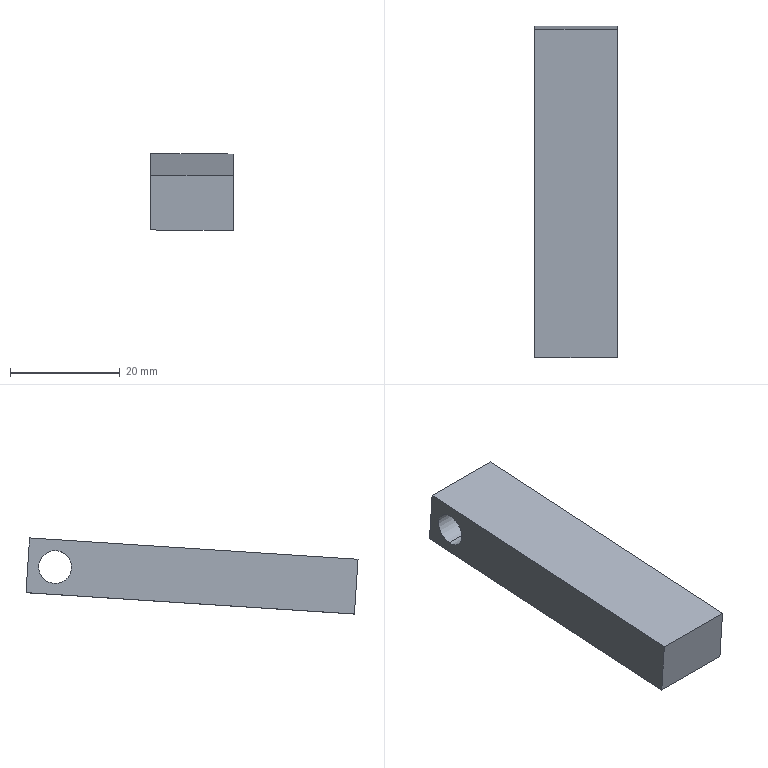Component | SolidWorks | ClampingPlate-1 | 1 solid | 8 faces | box 15.01 x 60.52 x 13.88 mm | volume 8576 mm3 | plane 6 | cylinder 2 | commonest cylinder face diameters 6 x2
build123d program:
from build123d import *

# Parameters (mm, degrees)
SKETCH1_W           = 60
SKETCH1_H           = 10
BOSS_EXTRUDE1_DEPTH = 15
SKETCH2_R           = 3
CUT_EXTRUDE1_DEPTH  = 20


with BuildPart() as part:
    # Sketch1 → Boss-Extrude1 (new body)
    with BuildSketch(Plane(origin=(0, 0, 0), x_dir=(1, 0, 0), z_dir=(0, 1, 0))):
        Rectangle(SKETCH1_W, SKETCH1_H)
    extrude(amount=BOSS_EXTRUDE1_DEPTH)

    # Sketch2 → Cut-Extrude1 (cut)
    with BuildSketch(Plane(origin=(0, 15, 0), x_dir=(1, 0, 0), z_dir=(0, 1, 0))):
        with Locations(Location((25, 0, 0), (0, 0, 270))):
            Circle(SKETCH2_R)
    extrude(amount=-CUT_EXTRUDE1_DEPTH, mode=Mode.SUBTRACT)


solid = part.part

# Placed as in the assembly
solid = solid.moved(Location((-132.643, 740.362, 1090.615), (3.717, 0.06177, 89.996)))
STEP:
#1=CARTESIAN_POINT('',(-5.222,30.123,43.119));
#2=VERTEX_POINT('',#1);
#3=CARTESIAN_POINT('',(-5.222,30.138,42.884));
#4=VERTEX_POINT('',#3);
#5=CARTESIAN_POINT('',(-5.222,30.13,43.001));
#6=DIRECTION('',(1.,0.,-0.00108));
#7=DIRECTION('',(-0.001078,0.06482,-0.9979));
#8=AXIS2_PLACEMENT_3D('',#5,#6,#7);
#9=CIRCLE('',#8,0.1181);
#10=EDGE_CURVE('',#2,#4,#9,.T.);
#11=ORIENTED_EDGE('',*,*,#10,.T.);
#12=CARTESIAN_POINT('',(-5.813,30.138,42.884));
#13=VERTEX_POINT('',#12);
#14=CARTESIAN_POINT('',(-5.025,30.138,42.883));
#15=DIRECTION('',(-1.,-0.,0.00108));
#16=VECTOR('',#15,39.37);
#17=LINE('',#14,#16);
#18=EDGE_CURVE('',#4,#13,#17,.T.);
#19=ORIENTED_EDGE('',*,*,#18,.T.);
#20=CARTESIAN_POINT('',(-5.813,30.123,43.12));
#21=VERTEX_POINT('',#20);
#22=CARTESIAN_POINT('',(-5.813,30.13,43.002));
#23=DIRECTION('',(-1.,-0.,0.00108));
#24=DIRECTION('',(0.001078,-0.06482,0.9979));
#25=AXIS2_PLACEMENT_3D('',#22,#23,#24);
#26=CIRCLE('',#25,0.1181);
#27=EDGE_CURVE('',#13,#21,#26,.T.);
#28=ORIENTED_EDGE('',*,*,#27,.T.);
#29=CARTESIAN_POINT('',(-5.025,30.123,43.119));
#30=DIRECTION('',(-1.,-0.,0.00108));
#31=VECTOR('',#30,39.37);
#32=LINE('',#29,#31);
#33=EDGE_CURVE('',#2,#21,#32,.T.);
#34=ORIENTED_EDGE('',*,*,#33,.F.);
#35=EDGE_LOOP('',(#11,#19,#28,#34));
#36=FACE_OUTER_BOUND('',#35,.T.);
#37=CARTESIAN_POINT('',(-5.025,30.13,43.001));
#38=DIRECTION('',(-1.,-0.,0.00108));
#39=DIRECTION('',(0.001078,-0.06482,0.9979));
#40=AXIS2_PLACEMENT_3D('',#37,#38,#39);
#41=CYLINDRICAL_SURFACE('',#40,0.1181);
#42=ADVANCED_FACE('',(#36),#41,.F.);
#43=CARTESIAN_POINT('',(-5.222,30.314,43.211));
#44=VERTEX_POINT('',#43);
#45=CARTESIAN_POINT('',(-5.222,30.339,42.818));
#46=VERTEX_POINT('',#45);
#47=CARTESIAN_POINT('',(-5.222,30.314,43.211));
#48=DIRECTION('',(-0.001078,0.06482,-0.9979));
#49=VECTOR('',#48,39.37);
#50=LINE('',#47,#49);
#51=EDGE_CURVE('',#44,#46,#50,.T.);
#52=ORIENTED_EDGE('',*,*,#51,.T.);
#53=CARTESIAN_POINT('',(-5.813,30.339,42.818));
#54=VERTEX_POINT('',#53);
#55=CARTESIAN_POINT('',(-5.813,30.339,42.818));
#56=DIRECTION('',(1.,0.,-0.00108));
#57=VECTOR('',#56,39.37);
#58=LINE('',#55,#57);
#59=EDGE_CURVE('',#54,#46,#58,.T.);
#60=ORIENTED_EDGE('',*,*,#59,.F.);
#61=CARTESIAN_POINT('',(-5.812,30.314,43.211));
#62=VERTEX_POINT('',#61);
#63=CARTESIAN_POINT('',(-5.812,30.314,43.211));
#64=DIRECTION('',(-0.001078,0.06482,-0.9979));
#65=VECTOR('',#64,39.37);
#66=LINE('',#63,#65);
#67=EDGE_CURVE('',#62,#54,#66,.T.);
#68=ORIENTED_EDGE('',*,*,#67,.F.);
#69=CARTESIAN_POINT('',(-5.812,30.314,43.211));
#70=DIRECTION('',(1.,0.,-0.00108));
#71=VECTOR('',#70,39.37);
#72=LINE('',#69,#71);
#73=EDGE_CURVE('',#62,#44,#72,.T.);
#74=ORIENTED_EDGE('',*,*,#73,.T.);
#75=EDGE_LOOP('',(#52,#60,#68,#74));
#76=FACE_OUTER_BOUND('',#75,.T.);
#77=CARTESIAN_POINT('',(-5.812,30.314,43.211));
#78=DIRECTION('',(-0.00007004,-0.9979,-0.06482));
#79=DIRECTION('',(0.001078,-0.06482,0.9979));
#80=AXIS2_PLACEMENT_3D('',#77,#78,#79);
#81=PLANE('',#80);
#82=ADVANCED_FACE('',(#76),#81,.F.);
#83=CARTESIAN_POINT('',(-5.222,27.982,42.665));
#84=VERTEX_POINT('',#83);
#85=CARTESIAN_POINT('',(-5.222,27.982,42.665));
#86=DIRECTION('',(-0.00007004,-0.9979,-0.06482));
#87=VECTOR('',#86,39.37);
#88=LINE('',#85,#87);
#89=EDGE_CURVE('',#46,#84,#88,.T.);
#90=ORIENTED_EDGE('',*,*,#89,.T.);
#91=CARTESIAN_POINT('',(-5.813,27.982,42.665));
#92=VERTEX_POINT('',#91);
#93=CARTESIAN_POINT('',(-5.813,27.982,42.665));
#94=DIRECTION('',(1.,0.,-0.00108));
#95=VECTOR('',#94,39.37);
#96=LINE('',#93,#95);
#97=EDGE_CURVE('',#92,#84,#96,.T.);
#98=ORIENTED_EDGE('',*,*,#97,.F.);
#99=CARTESIAN_POINT('',(-5.813,27.982,42.665));
#100=DIRECTION('',(-0.00007004,-0.9979,-0.06482));
#101=VECTOR('',#100,39.37);
#102=LINE('',#99,#101);
#103=EDGE_CURVE('',#54,#92,#102,.T.);
#104=ORIENTED_EDGE('',*,*,#103,.F.);
#105=ORIENTED_EDGE('',*,*,#59,.T.);
#106=EDGE_LOOP('',(#90,#98,#104,#105));
#107=FACE_OUTER_BOUND('',#106,.T.);
#108=CARTESIAN_POINT('',(-5.813,27.982,42.665));
#109=DIRECTION('',(0.001078,-0.06482,0.9979));
#110=DIRECTION('',(0.00007004,0.9979,0.06482));
#111=AXIS2_PLACEMENT_3D('',#108,#109,#110);
#112=PLANE('',#111);
#113=ADVANCED_FACE('',(#107),#112,.F.);
#114=CARTESIAN_POINT('',(-5.222,27.957,43.057));
#115=VERTEX_POINT('',#114);
#116=CARTESIAN_POINT('',(-5.222,27.957,43.057));
#117=DIRECTION('',(0.001078,-0.06482,0.9979));
#118=VECTOR('',#117,39.37);
#119=LINE('',#116,#118);
#120=EDGE_CURVE('',#84,#115,#119,.T.);
#121=ORIENTED_EDGE('',*,*,#120,.T.);
#122=CARTESIAN_POINT('',(-5.813,27.957,43.058));
#123=VERTEX_POINT('',#122);
#124=CARTESIAN_POINT('',(-5.813,27.957,43.058));
#125=DIRECTION('',(1.,0.,-0.00108));
#126=VECTOR('',#125,39.37);
#127=LINE('',#124,#126);
#128=EDGE_CURVE('',#123,#115,#127,.T.);
#129=ORIENTED_EDGE('',*,*,#128,.F.);
#130=CARTESIAN_POINT('',(-5.813,27.957,43.058));
#131=DIRECTION('',(0.001078,-0.06482,0.9979));
#132=VECTOR('',#131,39.37);
#133=LINE('',#130,#132);
#134=EDGE_CURVE('',#92,#123,#133,.T.);
#135=ORIENTED_EDGE('',*,*,#134,.F.);
#136=ORIENTED_EDGE('',*,*,#97,.T.);
#137=EDGE_LOOP('',(#121,#129,#135,#136));
#138=FACE_OUTER_BOUND('',#137,.T.);
#139=CARTESIAN_POINT('',(-5.813,27.957,43.058));
#140=DIRECTION('',(0.00007004,0.9979,0.06482));
#141=DIRECTION('',(-0.001078,0.06482,-0.9979));
#142=AXIS2_PLACEMENT_3D('',#139,#140,#141);
#143=PLANE('',#142);
#144=ADVANCED_FACE('',(#138),#143,.F.);
#145=CARTESIAN_POINT('',(-5.222,27.957,43.057));
#146=DIRECTION('',(0.00007004,0.9979,0.06482));
#147=VECTOR('',#146,39.37);
#148=LINE('',#145,#147);
#149=EDGE_CURVE('',#115,#44,#148,.T.);
#150=ORIENTED_EDGE('',*,*,#149,.T.);
#151=ORIENTED_EDGE('',*,*,#73,.F.);
#152=CARTESIAN_POINT('',(-5.813,27.957,43.058));
#153=DIRECTION('',(0.00007004,0.9979,0.06482));
#154=VECTOR('',#153,39.37);
#155=LINE('',#152,#154);
#156=EDGE_CURVE('',#123,#62,#155,.T.);
#157=ORIENTED_EDGE('',*,*,#156,.F.);
#158=ORIENTED_EDGE('',*,*,#128,.T.);
#159=EDGE_LOOP('',(#150,#151,#157,#158));
#160=FACE_OUTER_BOUND('',#159,.T.);
#161=CARTESIAN_POINT('',(-5.813,27.957,43.058));
#162=DIRECTION('',(-0.001078,0.06482,-0.9979));
#163=DIRECTION('',(-0.00007004,-0.9979,-0.06482));
#164=AXIS2_PLACEMENT_3D('',#161,#162,#163);
#165=PLANE('',#164);
#166=ADVANCED_FACE('',(#160),#165,.F.);
#167=CARTESIAN_POINT('',(-5.813,30.13,43.002));
#168=DIRECTION('',(-1.,-0.,0.00108));
#169=DIRECTION('',(0.001078,-0.06482,0.9979));
#170=AXIS2_PLACEMENT_3D('',#167,#168,#169);
#171=CIRCLE('',#170,0.1181);
#172=EDGE_CURVE('',#21,#13,#171,.T.);
#173=ORIENTED_EDGE('',*,*,#172,.F.);
#174=ORIENTED_EDGE('',*,*,#27,.F.);
#175=EDGE_LOOP('',(#173,#174));
#176=FACE_BOUND('',#175,.T.);
#177=ORIENTED_EDGE('',*,*,#67,.T.);
#178=ORIENTED_EDGE('',*,*,#103,.T.);
#179=ORIENTED_EDGE('',*,*,#134,.T.);
#180=ORIENTED_EDGE('',*,*,#156,.T.);
#181=EDGE_LOOP('',(#177,#178,#179,#180));
#182=FACE_OUTER_BOUND('',#181,.T.);
#183=CARTESIAN_POINT('',(-5.813,29.148,42.938));
#184=DIRECTION('',(1.,0.,-0.00108));
#185=DIRECTION('',(-0.001078,0.06482,-0.9979));
#186=AXIS2_PLACEMENT_3D('',#183,#184,#185);
#187=PLANE('',#186);
#188=ADVANCED_FACE('',(#176,#182),#187,.F.);
#189=ORIENTED_EDGE('',*,*,#10,.F.);
#190=CARTESIAN_POINT('',(-5.222,30.13,43.001));
#191=DIRECTION('',(1.,0.,-0.00108));
#192=DIRECTION('',(-0.001078,0.06482,-0.9979));
#193=AXIS2_PLACEMENT_3D('',#190,#191,#192);
#194=CIRCLE('',#193,0.1181);
#195=EDGE_CURVE('',#4,#2,#194,.T.);
#196=ORIENTED_EDGE('',*,*,#195,.F.);
#197=EDGE_LOOP('',(#189,#196));
#198=FACE_BOUND('',#197,.T.);
#199=ORIENTED_EDGE('',*,*,#51,.F.);
#200=ORIENTED_EDGE('',*,*,#149,.F.);
#201=ORIENTED_EDGE('',*,*,#120,.F.);
#202=ORIENTED_EDGE('',*,*,#89,.F.);
#203=EDGE_LOOP('',(#199,#200,#201,#202));
#204=FACE_OUTER_BOUND('',#203,.T.);
#205=CARTESIAN_POINT('',(-5.222,29.148,42.938));
#206=DIRECTION('',(1.,0.,-0.00108));
#207=DIRECTION('',(-0.001078,0.06482,-0.9979));
#208=AXIS2_PLACEMENT_3D('',#205,#206,#207);
#209=PLANE('',#208);
#210=ADVANCED_FACE('',(#198,#204),#209,.T.);
#211=ORIENTED_EDGE('',*,*,#18,.F.);
#212=ORIENTED_EDGE('',*,*,#195,.T.);
#213=ORIENTED_EDGE('',*,*,#33,.T.);
#214=ORIENTED_EDGE('',*,*,#172,.T.);
#215=EDGE_LOOP('',(#211,#212,#213,#214));
#216=FACE_OUTER_BOUND('',#215,.T.);
#217=CARTESIAN_POINT('',(-5.025,30.13,43.001));
#218=DIRECTION('',(-1.,-0.,0.00108));
#219=DIRECTION('',(0.001078,-0.06482,0.9979));
#220=AXIS2_PLACEMENT_3D('',#217,#218,#219);
#221=CYLINDRICAL_SURFACE('',#220,0.1181);
#222=ADVANCED_FACE('',(#216),#221,.F.);
#223=CLOSED_SHELL('',(#42,#82,#113,#144,#166,#188,#210,#222));
#224=MANIFOLD_SOLID_BREP('',#223);
#225=CARTESIAN_POINT('',(0.,0.,0.));
#226=DIRECTION('',(0.,0.,1.));
#227=DIRECTION('',(1.,0.,0.));
#228=AXIS2_PLACEMENT_3D('',#225,#226,#227);
#229=(LENGTH_UNIT()NAMED_UNIT(*)SI_UNIT($,.METRE.));
#230=LENGTH_MEASURE_WITH_UNIT(LENGTH_MEASURE(0.0254),#229);
#231=DIMENSIONAL_EXPONENTS(1.,0.,0.,0.,0.,0.,0.);
#232=(CONVERSION_BASED_UNIT('',#230)LENGTH_UNIT()NAMED_UNIT(#231));
#233=UNCERTAINTY_MEASURE_WITH_UNIT(LENGTH_MEASURE(0.00001),#232,'','');
#234=(NAMED_UNIT(*)PLANE_ANGLE_UNIT()SI_UNIT($,.RADIAN.));
#235=(NAMED_UNIT(*)SI_UNIT($,.STERADIAN.)SOLID_ANGLE_UNIT());
#236=(GEOMETRIC_REPRESENTATION_CONTEXT(3)GLOBAL_UNCERTAINTY_ASSIGNED_CONTEXT((#233))GLOBAL_UNIT_ASSIGNED_CONTEXT((#232,#234,#235))REPRESENTATION_CONTEXT('',''));
#237=ADVANCED_BREP_SHAPE_REPRESENTATION('',(#224,#228),#236);
#238=COLOUR_RGB('',0.7922,0.8196,0.9333);
#239=FILL_AREA_STYLE_COLOUR('',#238);
#240=FILL_AREA_STYLE('',(#239));
#241=SURFACE_STYLE_FILL_AREA(#240);
#242=SURFACE_SIDE_STYLE('',(#241));
#243=SURFACE_STYLE_USAGE(.BOTH.,#242);
#244=PRESENTATION_STYLE_ASSIGNMENT((#243));
#245=STYLED_ITEM('',(#244),#224);
#246=PRESENTATION_LAYER_ASSIGNMENT('','',(#245));
#247=(LENGTH_UNIT()NAMED_UNIT(*)SI_UNIT($,.METRE.));
#248=LENGTH_MEASURE_WITH_UNIT(LENGTH_MEASURE(0.0254),#247);
#249=DIMENSIONAL_EXPONENTS(1.,0.,0.,0.,0.,0.,0.);
#250=(CONVERSION_BASED_UNIT('',#248)LENGTH_UNIT()NAMED_UNIT(#249));
#251=UNCERTAINTY_MEASURE_WITH_UNIT(LENGTH_MEASURE(0.00001),#250,'','');
#252=(NAMED_UNIT(*)PLANE_ANGLE_UNIT()SI_UNIT($,.RADIAN.));
#253=(NAMED_UNIT(*)SI_UNIT($,.STERADIAN.)SOLID_ANGLE_UNIT());
#254=(GEOMETRIC_REPRESENTATION_CONTEXT(3)GLOBAL_UNCERTAINTY_ASSIGNED_CONTEXT((#251))GLOBAL_UNIT_ASSIGNED_CONTEXT((#250,#252,#253))REPRESENTATION_CONTEXT('',''));
#255=MECHANICAL_DESIGN_GEOMETRIC_PRESENTATION_REPRESENTATION('',(#245),#254);